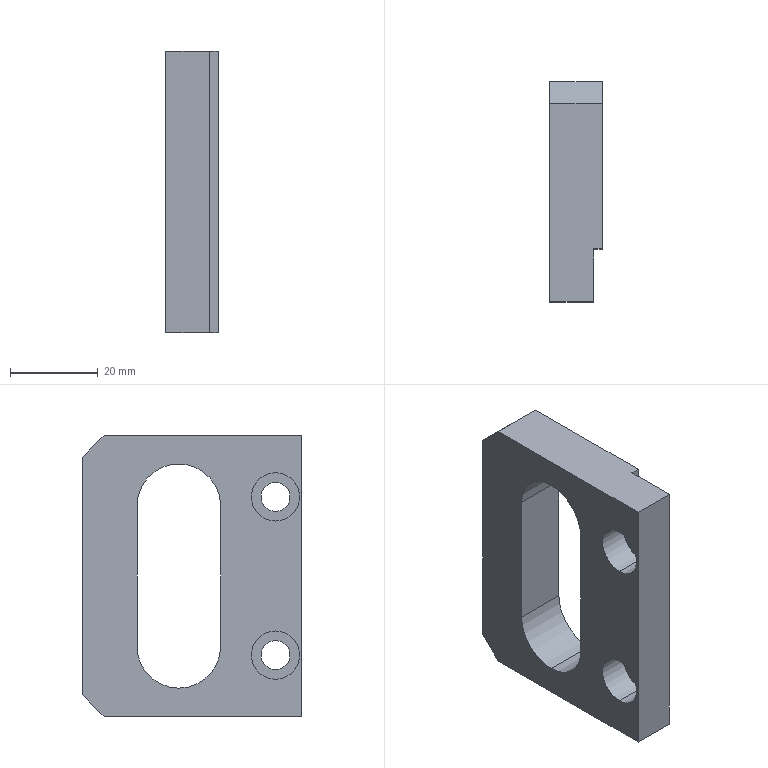Component | SolidWorks | ClampingAssembly-1_A76-1 | 1 solid | 25 faces | box 12 x 50 x 64 mm | volume 24339 mm3 | plane 14 | cylinder 11 | commonest cylinder face diameters 11 x4 6.6 x4 19.02 x3 | material S136
build123d program:
from build123d import *

# Parameters (mm, degrees)
SKETCH1_W                                          = 64
SKETCH1_H                                          = 50
BOSS_EXTRUDE1_DEPTH                                = 6
CUT_EXTRUDE1_DEPTH                                 = 43.344
CHAMFER1_SIZE                                      = 5
SKETCH3_W                                          = 64
SKETCH3_H                                          = 12
CUT_EXTRUDE2_DEPTH                                 = 2
HOLE_SIZE_ACCORDING_TO_TYPE_1_OF_HEXAG_D           = 6.6
HOLE_SIZE_ACCORDING_TO_TYPE_1_OF_HEXAG_CBORE_D     = 11
HOLE_SIZE_ACCORDING_TO_TYPE_1_OF_HEXAG_CBORE_DEPTH = 6.8


with BuildPart() as part:
    # Sketch1 → Boss-Extrude1 (new, symmetric)
    with BuildSketch(Plane(origin=(0, 0, 0), x_dir=(0, 0, -1), z_dir=(1, 0, 0))):
        Rectangle(SKETCH1_W, SKETCH1_H)
    extrude(amount=BOSS_EXTRUDE1_DEPTH, both=True)

    # Sketch2 → Cut-Extrude1 (cut, through all)
    with BuildSketch(Plane(origin=(6, 0, 0), x_dir=(0, 0, -1), z_dir=(1, 0, 0))):
        with BuildLine():
            Line((-16, 12.51), (16, 12.51))
            ThreePointArc((16, 12.51), (25.51, 3), (16, -6.51))
            Line((16, -6.51), (-16, -6.51))
            ThreePointArc((-16, -6.51), (-25.51, 3), (-16, 12.51))
        make_face()
    extrude(amount=-CUT_EXTRUDE1_DEPTH, mode=Mode.SUBTRACT)

    # Chamfer1
    chamfer1_edges = [part.edges().sort_by_distance(p)[0] for p in [
        (0, 25, 32),
        (0, 25, -32),
    ]]
    chamfer(chamfer1_edges, length=CHAMFER1_SIZE)

    # Sketch3 → Cut-Extrude2 (cut)
    with BuildSketch(Plane(origin=(6, 0, 0), x_dir=(0, 0, -1), z_dir=(1, 0, 0))):
        with Locations((0, -19)):
            Rectangle(SKETCH3_W, SKETCH3_H)
    extrude(amount=-CUT_EXTRUDE2_DEPTH, mode=Mode.SUBTRACT)

    # Hole Size _According to_ Type 1 of Hexag (through all)
    with Locations(Plane.ZY.offset(6)):
        with Locations((-18, -19), (18, -19)):
            CounterBoreHole(HOLE_SIZE_ACCORDING_TO_TYPE_1_OF_HEXAG_D / 2, HOLE_SIZE_ACCORDING_TO_TYPE_1_OF_HEXAG_CBORE_D / 2, HOLE_SIZE_ACCORDING_TO_TYPE_1_OF_HEXAG_CBORE_DEPTH)


solid = part.part

# Placed as in the assembly
solid = solid.moved(Location((-8.551, 63.036, -37.5), (0, 0, 0)))
STEP:
#1=COLOUR_RGB('',0.7922,0.8196,0.9333);
#2=FILL_AREA_STYLE_COLOUR('',#1);
#3=FILL_AREA_STYLE('',(#2));
#4=SURFACE_STYLE_FILL_AREA(#3);
#5=SURFACE_SIDE_STYLE('',(#4));
#6=SURFACE_STYLE_USAGE(.BOTH.,#5);
#7=PRESENTATION_STYLE_ASSIGNMENT((#6));
#8=CARTESIAN_POINT('',(-0.3051,1.734,-2.402));
#9=VERTEX_POINT('',#8);
#10=CARTESIAN_POINT('',(-0.3051,1.734,-1.969));
#11=VERTEX_POINT('',#10);
#12=CARTESIAN_POINT('',(-0.3051,1.734,-2.185));
#13=DIRECTION('',(-1.,0.,0.));
#14=DIRECTION('',(0.,0.,1.));
#15=AXIS2_PLACEMENT_3D('',#12,#13,#14);
#16=CIRCLE('',#15,0.2165);
#17=EDGE_CURVE('',#9,#11,#16,.T.);
#18=ORIENTED_EDGE('',*,*,#17,.F.);
#19=CARTESIAN_POINT('',(-0.5729,1.734,-2.402));
#20=VERTEX_POINT('',#19);
#21=CARTESIAN_POINT('',(-0.5729,1.734,-2.402));
#22=DIRECTION('',(-1.,0.,0.));
#23=VECTOR('',#22,39.37);
#24=LINE('',#21,#23);
#25=EDGE_CURVE('',#9,#20,#24,.T.);
#26=ORIENTED_EDGE('',*,*,#25,.T.);
#27=CARTESIAN_POINT('',(-0.5729,1.734,-1.969));
#28=VERTEX_POINT('',#27);
#29=CARTESIAN_POINT('',(-0.5729,1.734,-2.185));
#30=DIRECTION('',(-1.,0.,0.));
#31=DIRECTION('',(0.,0.,1.));
#32=AXIS2_PLACEMENT_3D('',#29,#30,#31);
#33=CIRCLE('',#32,0.2165);
#34=EDGE_CURVE('',#20,#28,#33,.T.);
#35=ORIENTED_EDGE('',*,*,#34,.T.);
#36=CARTESIAN_POINT('',(-0.5729,1.734,-1.969));
#37=DIRECTION('',(-1.,0.,0.));
#38=VECTOR('',#37,39.37);
#39=LINE('',#36,#38);
#40=EDGE_CURVE('',#11,#28,#39,.T.);
#41=ORIENTED_EDGE('',*,*,#40,.F.);
#42=EDGE_LOOP('',(#18,#26,#35,#41));
#43=FACE_OUTER_BOUND('',#42,.T.);
#44=CARTESIAN_POINT('',(-0.5729,1.734,-2.185));
#45=DIRECTION('',(-1.,0.,0.));
#46=DIRECTION('',(0.,0.,1.));
#47=AXIS2_PLACEMENT_3D('',#44,#45,#46);
#48=CYLINDRICAL_SURFACE('',#47,0.2165);
#49=ADVANCED_FACE('',(#43),#48,.F.);
#50=CARTESIAN_POINT('',(-0.1792,1.734,-2.315));
#51=VERTEX_POINT('',#50);
#52=CARTESIAN_POINT('',(-0.1792,1.734,-2.055));
#53=VERTEX_POINT('',#52);
#54=CARTESIAN_POINT('',(-0.1792,1.734,-2.185));
#55=DIRECTION('',(-1.,0.,0.));
#56=DIRECTION('',(0.,0.,1.));
#57=AXIS2_PLACEMENT_3D('',#54,#55,#56);
#58=CIRCLE('',#57,0.1299);
#59=EDGE_CURVE('',#51,#53,#58,.T.);
#60=ORIENTED_EDGE('',*,*,#59,.F.);
#61=CARTESIAN_POINT('',(-0.3051,1.734,-2.315));
#62=VERTEX_POINT('',#61);
#63=CARTESIAN_POINT('',(-0.5729,1.734,-2.315));
#64=DIRECTION('',(-1.,0.,0.));
#65=VECTOR('',#64,39.37);
#66=LINE('',#63,#65);
#67=EDGE_CURVE('',#51,#62,#66,.T.);
#68=ORIENTED_EDGE('',*,*,#67,.T.);
#69=CARTESIAN_POINT('',(-0.3051,1.734,-2.055));
#70=VERTEX_POINT('',#69);
#71=CARTESIAN_POINT('',(-0.3051,1.734,-2.185));
#72=DIRECTION('',(-1.,0.,0.));
#73=DIRECTION('',(0.,0.,1.));
#74=AXIS2_PLACEMENT_3D('',#71,#72,#73);
#75=CIRCLE('',#74,0.1299);
#76=EDGE_CURVE('',#62,#70,#75,.T.);
#77=ORIENTED_EDGE('',*,*,#76,.T.);
#78=CARTESIAN_POINT('',(-0.5729,1.734,-2.055));
#79=DIRECTION('',(-1.,0.,0.));
#80=VECTOR('',#79,39.37);
#81=LINE('',#78,#80);
#82=EDGE_CURVE('',#53,#70,#81,.T.);
#83=ORIENTED_EDGE('',*,*,#82,.F.);
#84=EDGE_LOOP('',(#60,#68,#77,#83));
#85=FACE_OUTER_BOUND('',#84,.T.);
#86=CARTESIAN_POINT('',(-0.5729,1.734,-2.185));
#87=DIRECTION('',(-1.,0.,0.));
#88=DIRECTION('',(0.,0.,1.));
#89=AXIS2_PLACEMENT_3D('',#86,#87,#88);
#90=CYLINDRICAL_SURFACE('',#89,0.1299);
#91=ADVANCED_FACE('',(#85),#90,.F.);
#92=CARTESIAN_POINT('',(-0.3051,1.734,-0.9843));
#93=VERTEX_POINT('',#92);
#94=CARTESIAN_POINT('',(-0.3051,1.734,-0.5512));
#95=VERTEX_POINT('',#94);
#96=CARTESIAN_POINT('',(-0.3051,1.734,-0.7677));
#97=DIRECTION('',(-1.,0.,0.));
#98=DIRECTION('',(0.,0.,1.));
#99=AXIS2_PLACEMENT_3D('',#96,#97,#98);
#100=CIRCLE('',#99,0.2165);
#101=EDGE_CURVE('',#93,#95,#100,.T.);
#102=ORIENTED_EDGE('',*,*,#101,.F.);
#103=CARTESIAN_POINT('',(-0.5729,1.734,-0.9843));
#104=VERTEX_POINT('',#103);
#105=CARTESIAN_POINT('',(-0.5729,1.734,-0.9843));
#106=DIRECTION('',(-1.,0.,0.));
#107=VECTOR('',#106,39.37);
#108=LINE('',#105,#107);
#109=EDGE_CURVE('',#93,#104,#108,.T.);
#110=ORIENTED_EDGE('',*,*,#109,.T.);
#111=CARTESIAN_POINT('',(-0.5729,1.734,-0.5512));
#112=VERTEX_POINT('',#111);
#113=CARTESIAN_POINT('',(-0.5729,1.734,-0.7677));
#114=DIRECTION('',(-1.,0.,0.));
#115=DIRECTION('',(0.,0.,1.));
#116=AXIS2_PLACEMENT_3D('',#113,#114,#115);
#117=CIRCLE('',#116,0.2165);
#118=EDGE_CURVE('',#104,#112,#117,.T.);
#119=ORIENTED_EDGE('',*,*,#118,.T.);
#120=CARTESIAN_POINT('',(-0.5729,1.734,-0.5512));
#121=DIRECTION('',(-1.,0.,0.));
#122=VECTOR('',#121,39.37);
#123=LINE('',#120,#122);
#124=EDGE_CURVE('',#95,#112,#123,.T.);
#125=ORIENTED_EDGE('',*,*,#124,.F.);
#126=EDGE_LOOP('',(#102,#110,#119,#125));
#127=FACE_OUTER_BOUND('',#126,.T.);
#128=CARTESIAN_POINT('',(-0.5729,1.734,-0.7677));
#129=DIRECTION('',(-1.,0.,0.));
#130=DIRECTION('',(0.,0.,1.));
#131=AXIS2_PLACEMENT_3D('',#128,#129,#130);
#132=CYLINDRICAL_SURFACE('',#131,0.2165);
#133=ADVANCED_FACE('',(#127),#132,.F.);
#134=CARTESIAN_POINT('',(-0.1792,1.734,-0.8976));
#135=VERTEX_POINT('',#134);
#136=CARTESIAN_POINT('',(-0.1792,1.734,-0.6378));
#137=VERTEX_POINT('',#136);
#138=CARTESIAN_POINT('',(-0.1792,1.734,-0.7677));
#139=DIRECTION('',(-1.,0.,0.));
#140=DIRECTION('',(0.,0.,1.));
#141=AXIS2_PLACEMENT_3D('',#138,#139,#140);
#142=CIRCLE('',#141,0.1299);
#143=EDGE_CURVE('',#135,#137,#142,.T.);
#144=ORIENTED_EDGE('',*,*,#143,.F.);
#145=CARTESIAN_POINT('',(-0.3051,1.734,-0.8976));
#146=VERTEX_POINT('',#145);
#147=CARTESIAN_POINT('',(-0.5729,1.734,-0.8976));
#148=DIRECTION('',(-1.,0.,0.));
#149=VECTOR('',#148,39.37);
#150=LINE('',#147,#149);
#151=EDGE_CURVE('',#135,#146,#150,.T.);
#152=ORIENTED_EDGE('',*,*,#151,.T.);
#153=CARTESIAN_POINT('',(-0.3051,1.734,-0.6378));
#154=VERTEX_POINT('',#153);
#155=CARTESIAN_POINT('',(-0.3051,1.734,-0.7677));
#156=DIRECTION('',(-1.,0.,0.));
#157=DIRECTION('',(0.,0.,1.));
#158=AXIS2_PLACEMENT_3D('',#155,#156,#157);
#159=CIRCLE('',#158,0.1299);
#160=EDGE_CURVE('',#146,#154,#159,.T.);
#161=ORIENTED_EDGE('',*,*,#160,.T.);
#162=CARTESIAN_POINT('',(-0.5729,1.734,-0.6378));
#163=DIRECTION('',(-1.,0.,0.));
#164=VECTOR('',#163,39.37);
#165=LINE('',#162,#164);
#166=EDGE_CURVE('',#137,#154,#165,.T.);
#167=ORIENTED_EDGE('',*,*,#166,.F.);
#168=EDGE_LOOP('',(#144,#152,#161,#167));
#169=FACE_OUTER_BOUND('',#168,.T.);
#170=CARTESIAN_POINT('',(-0.5729,1.734,-0.7677));
#171=DIRECTION('',(-1.,0.,0.));
#172=DIRECTION('',(0.,0.,1.));
#173=AXIS2_PLACEMENT_3D('',#170,#171,#172);
#174=CYLINDRICAL_SURFACE('',#173,0.1299);
#175=ADVANCED_FACE('',(#169),#174,.F.);
#176=CARTESIAN_POINT('',(-0.5729,2.6,-2.481));
#177=VERTEX_POINT('',#176);
#178=CARTESIAN_POINT('',(-0.5729,2.974,-2.106));
#179=VERTEX_POINT('',#178);
#180=CARTESIAN_POINT('',(-0.5729,2.6,-2.106));
#181=DIRECTION('',(1.,0.,0.));
#182=DIRECTION('',(0.,0.,-1.));
#183=AXIS2_PLACEMENT_3D('',#180,#181,#182);
#184=CIRCLE('',#183,0.3744);
#185=EDGE_CURVE('',#177,#179,#184,.T.);
#186=ORIENTED_EDGE('',*,*,#185,.F.);
#187=CARTESIAN_POINT('',(-0.1004,2.6,-2.481));
#188=VERTEX_POINT('',#187);
#189=CARTESIAN_POINT('',(-0.5729,2.6,-2.481));
#190=DIRECTION('',(1.,0.,0.));
#191=VECTOR('',#190,39.37);
#192=LINE('',#189,#191);
#193=EDGE_CURVE('',#177,#188,#192,.T.);
#194=ORIENTED_EDGE('',*,*,#193,.T.);
#195=CARTESIAN_POINT('',(-0.1004,2.974,-2.106));
#196=VERTEX_POINT('',#195);
#197=CARTESIAN_POINT('',(-0.1004,2.6,-2.106));
#198=DIRECTION('',(1.,0.,0.));
#199=DIRECTION('',(0.,0.,-1.));
#200=AXIS2_PLACEMENT_3D('',#197,#198,#199);
#201=CIRCLE('',#200,0.3744);
#202=EDGE_CURVE('',#188,#196,#201,.T.);
#203=ORIENTED_EDGE('',*,*,#202,.T.);
#204=CARTESIAN_POINT('',(-0.5729,2.974,-2.106));
#205=DIRECTION('',(1.,0.,0.));
#206=VECTOR('',#205,39.37);
#207=LINE('',#204,#206);
#208=EDGE_CURVE('',#179,#196,#207,.T.);
#209=ORIENTED_EDGE('',*,*,#208,.F.);
#210=EDGE_LOOP('',(#186,#194,#203,#209));
#211=FACE_OUTER_BOUND('',#210,.T.);
#212=CARTESIAN_POINT('',(-0.5729,2.6,-2.106));
#213=DIRECTION('',(1.,0.,0.));
#214=DIRECTION('',(0.,0.,-1.));
#215=AXIS2_PLACEMENT_3D('',#212,#213,#214);
#216=CYLINDRICAL_SURFACE('',#215,0.3744);
#217=ADVANCED_FACE('',(#211),#216,.F.);
#218=CARTESIAN_POINT('',(-0.1004,1.97,-2.736));
#219=VERTEX_POINT('',#218);
#220=CARTESIAN_POINT('',(-0.1004,3.269,-2.736));
#221=VERTEX_POINT('',#220);
#222=CARTESIAN_POINT('',(-0.1004,3.466,-2.736));
#223=DIRECTION('',(0.,1.,0.));
#224=VECTOR('',#223,39.37);
#225=LINE('',#222,#224);
#226=EDGE_CURVE('',#219,#221,#225,.T.);
#227=ORIENTED_EDGE('',*,*,#226,.F.);
#228=CARTESIAN_POINT('',(-0.1792,1.97,-2.736));
#229=VERTEX_POINT('',#228);
#230=CARTESIAN_POINT('',(-0.1792,1.97,-2.736));
#231=DIRECTION('',(1.,0.,0.));
#232=VECTOR('',#231,39.37);
#233=LINE('',#230,#232);
#234=EDGE_CURVE('',#229,#219,#233,.T.);
#235=ORIENTED_EDGE('',*,*,#234,.F.);
#236=CARTESIAN_POINT('',(-0.1792,1.497,-2.736));
#237=VERTEX_POINT('',#236);
#238=CARTESIAN_POINT('',(-0.1792,1.497,-2.736));
#239=DIRECTION('',(0.,1.,0.));
#240=VECTOR('',#239,39.37);
#241=LINE('',#238,#240);
#242=EDGE_CURVE('',#237,#229,#241,.T.);
#243=ORIENTED_EDGE('',*,*,#242,.F.);
#244=CARTESIAN_POINT('',(-0.5729,1.497,-2.736));
#245=VERTEX_POINT('',#244);
#246=CARTESIAN_POINT('',(-0.1004,1.497,-2.736));
#247=DIRECTION('',(-1.,0.,0.));
#248=VECTOR('',#247,39.37);
#249=LINE('',#246,#248);
#250=EDGE_CURVE('',#237,#245,#249,.T.);
#251=ORIENTED_EDGE('',*,*,#250,.T.);
#252=CARTESIAN_POINT('',(-0.5729,3.269,-2.736));
#253=VERTEX_POINT('',#252);
#254=CARTESIAN_POINT('',(-0.5729,3.466,-2.736));
#255=DIRECTION('',(0.,1.,0.));
#256=VECTOR('',#255,39.37);
#257=LINE('',#254,#256);
#258=EDGE_CURVE('',#245,#253,#257,.T.);
#259=ORIENTED_EDGE('',*,*,#258,.T.);
#260=CARTESIAN_POINT('',(-0.1004,3.269,-2.736));
#261=DIRECTION('',(1.,0.,0.));
#262=VECTOR('',#261,39.37);
#263=LINE('',#260,#262);
#264=EDGE_CURVE('',#253,#221,#263,.T.);
#265=ORIENTED_EDGE('',*,*,#264,.T.);
#266=EDGE_LOOP('',(#227,#235,#243,#251,#259,#265));
#267=FACE_OUTER_BOUND('',#266,.T.);
#268=CARTESIAN_POINT('',(-0.1004,3.466,-2.736));
#269=DIRECTION('',(0.,0.,1.));
#270=DIRECTION('',(1.,0.,0.));
#271=AXIS2_PLACEMENT_3D('',#268,#269,#270);
#272=PLANE('',#271);
#273=ADVANCED_FACE('',(#267),#272,.F.);
#274=CARTESIAN_POINT('',(-0.5729,3.466,-2.539));
#275=VERTEX_POINT('',#274);
#276=CARTESIAN_POINT('',(-0.5729,3.466,-0.4134));
#277=VERTEX_POINT('',#276);
#278=CARTESIAN_POINT('',(-0.5729,3.466,-0.2165));
#279=DIRECTION('',(0.,0.,1.));
#280=VECTOR('',#279,39.37);
#281=LINE('',#278,#280);
#282=EDGE_CURVE('',#275,#277,#281,.T.);
#283=ORIENTED_EDGE('',*,*,#282,.T.);
#284=CARTESIAN_POINT('',(-0.1004,3.466,-0.4134));
#285=VERTEX_POINT('',#284);
#286=CARTESIAN_POINT('',(-0.1004,3.466,-0.4134));
#287=DIRECTION('',(1.,0.,0.));
#288=VECTOR('',#287,39.37);
#289=LINE('',#286,#288);
#290=EDGE_CURVE('',#277,#285,#289,.T.);
#291=ORIENTED_EDGE('',*,*,#290,.T.);
#292=CARTESIAN_POINT('',(-0.1004,3.466,-2.539));
#293=VERTEX_POINT('',#292);
#294=CARTESIAN_POINT('',(-0.1004,3.466,-0.2165));
#295=DIRECTION('',(0.,0.,1.));
#296=VECTOR('',#295,39.37);
#297=LINE('',#294,#296);
#298=EDGE_CURVE('',#293,#285,#297,.T.);
#299=ORIENTED_EDGE('',*,*,#298,.F.);
#300=CARTESIAN_POINT('',(-0.1004,3.466,-2.539));
#301=DIRECTION('',(-1.,0.,0.));
#302=VECTOR('',#301,39.37);
#303=LINE('',#300,#302);
#304=EDGE_CURVE('',#293,#275,#303,.T.);
#305=ORIENTED_EDGE('',*,*,#304,.T.);
#306=EDGE_LOOP('',(#283,#291,#299,#305));
#307=FACE_OUTER_BOUND('',#306,.T.);
#308=CARTESIAN_POINT('',(-0.1004,3.466,-0.2165));
#309=DIRECTION('',(0.,-1.,0.));
#310=DIRECTION('',(0.,0.,-1.));
#311=AXIS2_PLACEMENT_3D('',#308,#309,#310);
#312=PLANE('',#311);
#313=ADVANCED_FACE('',(#307),#312,.F.);
#314=CARTESIAN_POINT('',(-0.1792,1.97,-0.2165));
#315=VERTEX_POINT('',#314);
#316=CARTESIAN_POINT('',(-0.1792,1.497,-0.2165));
#317=VERTEX_POINT('',#316);
#318=CARTESIAN_POINT('',(-0.1792,1.497,-0.2165));
#319=DIRECTION('',(0.,-1.,0.));
#320=VECTOR('',#319,39.37);
#321=LINE('',#318,#320);
#322=EDGE_CURVE('',#315,#317,#321,.T.);
#323=ORIENTED_EDGE('',*,*,#322,.F.);
#324=CARTESIAN_POINT('',(-0.1004,1.97,-0.2165));
#325=VERTEX_POINT('',#324);
#326=CARTESIAN_POINT('',(-0.1792,1.97,-0.2165));
#327=DIRECTION('',(1.,0.,0.));
#328=VECTOR('',#327,39.37);
#329=LINE('',#326,#328);
#330=EDGE_CURVE('',#315,#325,#329,.T.);
#331=ORIENTED_EDGE('',*,*,#330,.T.);
#332=CARTESIAN_POINT('',(-0.1004,3.269,-0.2165));
#333=VERTEX_POINT('',#332);
#334=CARTESIAN_POINT('',(-0.1004,3.466,-0.2165));
#335=DIRECTION('',(0.,-1.,-0.));
#336=VECTOR('',#335,39.37);
#337=LINE('',#334,#336);
#338=EDGE_CURVE('',#333,#325,#337,.T.);
#339=ORIENTED_EDGE('',*,*,#338,.F.);
#340=CARTESIAN_POINT('',(-0.5729,3.269,-0.2165));
#341=VERTEX_POINT('',#340);
#342=CARTESIAN_POINT('',(-0.1004,3.269,-0.2165));
#343=DIRECTION('',(-1.,0.,0.));
#344=VECTOR('',#343,39.37);
#345=LINE('',#342,#344);
#346=EDGE_CURVE('',#333,#341,#345,.T.);
#347=ORIENTED_EDGE('',*,*,#346,.T.);
#348=CARTESIAN_POINT('',(-0.5729,1.497,-0.2165));
#349=VERTEX_POINT('',#348);
#350=CARTESIAN_POINT('',(-0.5729,3.466,-0.2165));
#351=DIRECTION('',(0.,-1.,-0.));
#352=VECTOR('',#351,39.37);
#353=LINE('',#350,#352);
#354=EDGE_CURVE('',#341,#349,#353,.T.);
#355=ORIENTED_EDGE('',*,*,#354,.T.);
#356=CARTESIAN_POINT('',(-0.1004,1.497,-0.2165));
#357=DIRECTION('',(-1.,0.,0.));
#358=VECTOR('',#357,39.37);
#359=LINE('',#356,#358);
#360=EDGE_CURVE('',#317,#349,#359,.T.);
#361=ORIENTED_EDGE('',*,*,#360,.F.);
#362=EDGE_LOOP('',(#323,#331,#339,#347,#355,#361));
#363=FACE_OUTER_BOUND('',#362,.T.);
#364=CARTESIAN_POINT('',(-0.1004,3.466,-0.2165));
#365=DIRECTION('',(0.,0.,-1.));
#366=DIRECTION('',(0.,1.,0.));
#367=AXIS2_PLACEMENT_3D('',#364,#365,#366);
#368=PLANE('',#367);
#369=ADVANCED_FACE('',(#363),#368,.F.);
#370=ORIENTED_EDGE('',*,*,#250,.F.);
#371=CARTESIAN_POINT('',(-0.1792,1.497,-0.2165));
#372=DIRECTION('',(0.,0.,-1.));
#373=VECTOR('',#372,39.37);
#374=LINE('',#371,#373);
#375=EDGE_CURVE('',#317,#237,#374,.T.);
#376=ORIENTED_EDGE('',*,*,#375,.F.);
#377=ORIENTED_EDGE('',*,*,#360,.T.);
#378=CARTESIAN_POINT('',(-0.5729,1.497,-0.2165));
#379=DIRECTION('',(0.,0.,-1.));
#380=VECTOR('',#379,39.37);
#381=LINE('',#378,#380);
#382=EDGE_CURVE('',#349,#245,#381,.T.);
#383=ORIENTED_EDGE('',*,*,#382,.T.);
#384=EDGE_LOOP('',(#370,#376,#377,#383));
#385=FACE_OUTER_BOUND('',#384,.T.);
#386=CARTESIAN_POINT('',(-0.1004,1.497,-0.2165));
#387=DIRECTION('',(0.,1.,0.));
#388=DIRECTION('',(0.,0.,1.));
#389=AXIS2_PLACEMENT_3D('',#386,#387,#388);
#390=PLANE('',#389);
#391=ADVANCED_FACE('',(#385),#390,.F.);
#392=CARTESIAN_POINT('',(-0.1004,1.97,-0.2165));
#393=DIRECTION('',(0.,0.,1.));
#394=VECTOR('',#393,39.37);
#395=LINE('',#392,#394);
#396=EDGE_CURVE('',#219,#325,#395,.T.);
#397=ORIENTED_EDGE('',*,*,#396,.F.);
#398=ORIENTED_EDGE('',*,*,#226,.T.);
#399=CARTESIAN_POINT('',(-0.1004,3.505,-2.5));
#400=DIRECTION('',(0.,0.7071,0.7071));
#401=VECTOR('',#400,39.37);
#402=LINE('',#399,#401);
#403=EDGE_CURVE('',#221,#293,#402,.T.);
#404=ORIENTED_EDGE('',*,*,#403,.T.);
#405=ORIENTED_EDGE('',*,*,#298,.T.);
#406=CARTESIAN_POINT('',(-0.1004,3.505,-0.4528));
#407=DIRECTION('',(0.,-0.7071,0.7071));
#408=VECTOR('',#407,39.37);
#409=LINE('',#406,#408);
#410=EDGE_CURVE('',#285,#333,#409,.T.);
#411=ORIENTED_EDGE('',*,*,#410,.T.);
#412=ORIENTED_EDGE('',*,*,#338,.T.);
#413=EDGE_LOOP('',(#397,#398,#404,#405,#411,#412));
#414=FACE_OUTER_BOUND('',#413,.T.);
#415=CARTESIAN_POINT('',(-0.1004,2.974,-0.8465));
#416=VERTEX_POINT('',#415);
#417=CARTESIAN_POINT('',(-0.1004,2.225,-0.8465));
#418=VERTEX_POINT('',#417);
#419=CARTESIAN_POINT('',(-0.1004,2.6,-0.8465));
#420=DIRECTION('',(1.,0.,0.));
#421=DIRECTION('',(0.,0.,-1.));
#422=AXIS2_PLACEMENT_3D('',#419,#420,#421);
#423=CIRCLE('',#422,0.3744);
#424=EDGE_CURVE('',#416,#418,#423,.T.);
#425=ORIENTED_EDGE('',*,*,#424,.F.);
#426=CARTESIAN_POINT('',(-0.1004,2.974,-0.8465));
#427=DIRECTION('',(0.,0.,1.));
#428=VECTOR('',#427,39.37);
#429=LINE('',#426,#428);
#430=EDGE_CURVE('',#196,#416,#429,.T.);
#431=ORIENTED_EDGE('',*,*,#430,.F.);
#432=ORIENTED_EDGE('',*,*,#202,.F.);
#433=CARTESIAN_POINT('',(-0.1004,2.225,-2.106));
#434=VERTEX_POINT('',#433);
#435=CARTESIAN_POINT('',(-0.1004,2.6,-2.106));
#436=DIRECTION('',(1.,0.,0.));
#437=DIRECTION('',(0.,0.,-1.));
#438=AXIS2_PLACEMENT_3D('',#435,#436,#437);
#439=CIRCLE('',#438,0.3744);
#440=EDGE_CURVE('',#434,#188,#439,.T.);
#441=ORIENTED_EDGE('',*,*,#440,.F.);
#442=CARTESIAN_POINT('',(-0.1004,2.225,-0.8465));
#443=DIRECTION('',(0.,0.,-1.));
#444=VECTOR('',#443,39.37);
#445=LINE('',#442,#444);
#446=EDGE_CURVE('',#418,#434,#445,.T.);
#447=ORIENTED_EDGE('',*,*,#446,.F.);
#448=EDGE_LOOP('',(#425,#431,#432,#441,#447));
#449=FACE_BOUND('',#448,.T.);
#450=CARTESIAN_POINT('',(-0.1004,2.482,-1.476));
#451=DIRECTION('',(1.,0.,0.));
#452=DIRECTION('',(0.,0.,-1.));
#453=AXIS2_PLACEMENT_3D('',#450,#451,#452);
#454=PLANE('',#453);
#455=ADVANCED_FACE('',(#414,#449),#454,.T.);
#456=CARTESIAN_POINT('',(-0.5729,1.734,-2.185));
#457=DIRECTION('',(-1.,0.,0.));
#458=DIRECTION('',(0.,0.,1.));
#459=AXIS2_PLACEMENT_3D('',#456,#457,#458);
#460=CIRCLE('',#459,0.2165);
#461=EDGE_CURVE('',#28,#20,#460,.T.);
#462=ORIENTED_EDGE('',*,*,#461,.F.);
#463=ORIENTED_EDGE('',*,*,#34,.F.);
#464=EDGE_LOOP('',(#462,#463));
#465=FACE_BOUND('',#464,.T.);
#466=CARTESIAN_POINT('',(-0.5729,1.734,-0.7677));
#467=DIRECTION('',(-1.,0.,0.));
#468=DIRECTION('',(0.,0.,1.));
#469=AXIS2_PLACEMENT_3D('',#466,#467,#468);
#470=CIRCLE('',#469,0.2165);
#471=EDGE_CURVE('',#112,#104,#470,.T.);
#472=ORIENTED_EDGE('',*,*,#471,.F.);
#473=ORIENTED_EDGE('',*,*,#118,.F.);
#474=EDGE_LOOP('',(#472,#473));
#475=FACE_BOUND('',#474,.T.);
#476=CARTESIAN_POINT('',(-0.5729,2.974,-0.8465));
#477=VERTEX_POINT('',#476);
#478=CARTESIAN_POINT('',(-0.5729,2.974,-0.8465));
#479=DIRECTION('',(0.,0.,1.));
#480=VECTOR('',#479,39.37);
#481=LINE('',#478,#480);
#482=EDGE_CURVE('',#179,#477,#481,.T.);
#483=ORIENTED_EDGE('',*,*,#482,.T.);
#484=CARTESIAN_POINT('',(-0.5729,2.225,-0.8465));
#485=VERTEX_POINT('',#484);
#486=CARTESIAN_POINT('',(-0.5729,2.6,-0.8465));
#487=DIRECTION('',(1.,0.,0.));
#488=DIRECTION('',(0.,0.,-1.));
#489=AXIS2_PLACEMENT_3D('',#486,#487,#488);
#490=CIRCLE('',#489,0.3744);
#491=EDGE_CURVE('',#477,#485,#490,.T.);
#492=ORIENTED_EDGE('',*,*,#491,.T.);
#493=CARTESIAN_POINT('',(-0.5729,2.225,-2.106));
#494=VERTEX_POINT('',#493);
#495=CARTESIAN_POINT('',(-0.5729,2.225,-0.8465));
#496=DIRECTION('',(0.,0.,-1.));
#497=VECTOR('',#496,39.37);
#498=LINE('',#495,#497);
#499=EDGE_CURVE('',#485,#494,#498,.T.);
#500=ORIENTED_EDGE('',*,*,#499,.T.);
#501=CARTESIAN_POINT('',(-0.5729,2.6,-2.106));
#502=DIRECTION('',(1.,0.,0.));
#503=DIRECTION('',(0.,0.,-1.));
#504=AXIS2_PLACEMENT_3D('',#501,#502,#503);
#505=CIRCLE('',#504,0.3744);
#506=EDGE_CURVE('',#494,#177,#505,.T.);
#507=ORIENTED_EDGE('',*,*,#506,.T.);
#508=ORIENTED_EDGE('',*,*,#185,.T.);
#509=EDGE_LOOP('',(#483,#492,#500,#507,#508));
#510=FACE_BOUND('',#509,.T.);
#511=ORIENTED_EDGE('',*,*,#354,.F.);
#512=CARTESIAN_POINT('',(-0.5729,3.269,-0.2165));
#513=DIRECTION('',(0.,0.7071,-0.7071));
#514=VECTOR('',#513,39.37);
#515=LINE('',#512,#514);
#516=EDGE_CURVE('',#341,#277,#515,.T.);
#517=ORIENTED_EDGE('',*,*,#516,.T.);
#518=ORIENTED_EDGE('',*,*,#282,.F.);
#519=CARTESIAN_POINT('',(-0.5729,3.466,-2.539));
#520=DIRECTION('',(0.,-0.7071,-0.7071));
#521=VECTOR('',#520,39.37);
#522=LINE('',#519,#521);
#523=EDGE_CURVE('',#275,#253,#522,.T.);
#524=ORIENTED_EDGE('',*,*,#523,.T.);
#525=ORIENTED_EDGE('',*,*,#258,.F.);
#526=ORIENTED_EDGE('',*,*,#382,.F.);
#527=EDGE_LOOP('',(#511,#517,#518,#524,#525,#526));
#528=FACE_OUTER_BOUND('',#527,.T.);
#529=CARTESIAN_POINT('',(-0.5729,2.482,-1.476));
#530=DIRECTION('',(1.,0.,0.));
#531=DIRECTION('',(0.,0.,-1.));
#532=AXIS2_PLACEMENT_3D('',#529,#530,#531);
#533=PLANE('',#532);
#534=ADVANCED_FACE('',(#465,#475,#510,#528),#533,.F.);
#535=ORIENTED_EDGE('',*,*,#424,.T.);
#536=CARTESIAN_POINT('',(-0.5729,2.225,-0.8465));
#537=DIRECTION('',(1.,0.,0.));
#538=VECTOR('',#537,39.37);
#539=LINE('',#536,#538);
#540=EDGE_CURVE('',#485,#418,#539,.T.);
#541=ORIENTED_EDGE('',*,*,#540,.F.);
#542=ORIENTED_EDGE('',*,*,#491,.F.);
#543=CARTESIAN_POINT('',(-0.5729,2.974,-0.8465));
#544=DIRECTION('',(1.,0.,0.));
#545=VECTOR('',#544,39.37);
#546=LINE('',#543,#545);
#547=EDGE_CURVE('',#477,#416,#546,.T.);
#548=ORIENTED_EDGE('',*,*,#547,.T.);
#549=EDGE_LOOP('',(#535,#541,#542,#548));
#550=FACE_OUTER_BOUND('',#549,.T.);
#551=CARTESIAN_POINT('',(-0.5729,2.6,-0.8465));
#552=DIRECTION('',(1.,0.,0.));
#553=DIRECTION('',(0.,0.,-1.));
#554=AXIS2_PLACEMENT_3D('',#551,#552,#553);
#555=CYLINDRICAL_SURFACE('',#554,0.3744);
#556=ADVANCED_FACE('',(#550),#555,.F.);
#557=ORIENTED_EDGE('',*,*,#430,.T.);
#558=ORIENTED_EDGE('',*,*,#547,.F.);
#559=ORIENTED_EDGE('',*,*,#482,.F.);
#560=ORIENTED_EDGE('',*,*,#208,.T.);
#561=EDGE_LOOP('',(#557,#558,#559,#560));
#562=FACE_OUTER_BOUND('',#561,.T.);
#563=CARTESIAN_POINT('',(-0.5729,2.974,-0.8465));
#564=DIRECTION('',(0.,1.,0.));
#565=DIRECTION('',(0.,0.,1.));
#566=AXIS2_PLACEMENT_3D('',#563,#564,#565);
#567=PLANE('',#566);
#568=ADVANCED_FACE('',(#562),#567,.F.);
#569=ORIENTED_EDGE('',*,*,#193,.F.);
#570=ORIENTED_EDGE('',*,*,#506,.F.);
#571=CARTESIAN_POINT('',(-0.5729,2.225,-2.106));
#572=DIRECTION('',(1.,0.,0.));
#573=VECTOR('',#572,39.37);
#574=LINE('',#571,#573);
#575=EDGE_CURVE('',#494,#434,#574,.T.);
#576=ORIENTED_EDGE('',*,*,#575,.T.);
#577=ORIENTED_EDGE('',*,*,#440,.T.);
#578=EDGE_LOOP('',(#569,#570,#576,#577));
#579=FACE_OUTER_BOUND('',#578,.T.);
#580=CARTESIAN_POINT('',(-0.5729,2.6,-2.106));
#581=DIRECTION('',(1.,0.,0.));
#582=DIRECTION('',(0.,0.,-1.));
#583=AXIS2_PLACEMENT_3D('',#580,#581,#582);
#584=CYLINDRICAL_SURFACE('',#583,0.3744);
#585=ADVANCED_FACE('',(#579),#584,.F.);
#586=ORIENTED_EDGE('',*,*,#446,.T.);
#587=ORIENTED_EDGE('',*,*,#575,.F.);
#588=ORIENTED_EDGE('',*,*,#499,.F.);
#589=ORIENTED_EDGE('',*,*,#540,.T.);
#590=EDGE_LOOP('',(#586,#587,#588,#589));
#591=FACE_OUTER_BOUND('',#590,.T.);
#592=CARTESIAN_POINT('',(-0.5729,2.225,-0.8465));
#593=DIRECTION('',(0.,-1.,0.));
#594=DIRECTION('',(0.,0.,-1.));
#595=AXIS2_PLACEMENT_3D('',#592,#593,#594);
#596=PLANE('',#595);
#597=ADVANCED_FACE('',(#591),#596,.F.);
#598=ORIENTED_EDGE('',*,*,#410,.F.);
#599=ORIENTED_EDGE('',*,*,#290,.F.);
#600=ORIENTED_EDGE('',*,*,#516,.F.);
#601=ORIENTED_EDGE('',*,*,#346,.F.);
#602=EDGE_LOOP('',(#598,#599,#600,#601));
#603=FACE_OUTER_BOUND('',#602,.T.);
#604=CARTESIAN_POINT('',(-0.1004,3.269,-0.2165));
#605=DIRECTION('',(0.,-0.7071,-0.7071));
#606=DIRECTION('',(-1.,0.,0.));
#607=AXIS2_PLACEMENT_3D('',#604,#605,#606);
#608=PLANE('',#607);
#609=ADVANCED_FACE('',(#603),#608,.F.);
#610=ORIENTED_EDGE('',*,*,#403,.F.);
#611=ORIENTED_EDGE('',*,*,#264,.F.);
#612=ORIENTED_EDGE('',*,*,#523,.F.);
#613=ORIENTED_EDGE('',*,*,#304,.F.);
#614=EDGE_LOOP('',(#610,#611,#612,#613));
#615=FACE_OUTER_BOUND('',#614,.T.);
#616=CARTESIAN_POINT('',(-0.1004,3.466,-2.539));
#617=DIRECTION('',(0.,-0.7071,0.7071));
#618=DIRECTION('',(-1.,0.,0.));
#619=AXIS2_PLACEMENT_3D('',#616,#617,#618);
#620=PLANE('',#619);
#621=ADVANCED_FACE('',(#615),#620,.F.);
#622=ORIENTED_EDGE('',*,*,#396,.T.);
#623=ORIENTED_EDGE('',*,*,#330,.F.);
#624=CARTESIAN_POINT('',(-0.1792,1.97,-0.2165));
#625=DIRECTION('',(0.,0.,1.));
#626=VECTOR('',#625,39.37);
#627=LINE('',#624,#626);
#628=EDGE_CURVE('',#229,#315,#627,.T.);
#629=ORIENTED_EDGE('',*,*,#628,.F.);
#630=ORIENTED_EDGE('',*,*,#234,.T.);
#631=EDGE_LOOP('',(#622,#623,#629,#630));
#632=FACE_OUTER_BOUND('',#631,.T.);
#633=CARTESIAN_POINT('',(-0.1792,1.97,-0.2165));
#634=DIRECTION('',(0.,1.,0.));
#635=DIRECTION('',(0.,0.,1.));
#636=AXIS2_PLACEMENT_3D('',#633,#634,#635);
#637=PLANE('',#636);
#638=ADVANCED_FACE('',(#632),#637,.F.);
#639=CARTESIAN_POINT('',(-0.1792,1.734,-2.185));
#640=DIRECTION('',(-1.,0.,0.));
#641=DIRECTION('',(0.,0.,1.));
#642=AXIS2_PLACEMENT_3D('',#639,#640,#641);
#643=CIRCLE('',#642,0.1299);
#644=EDGE_CURVE('',#53,#51,#643,.T.);
#645=ORIENTED_EDGE('',*,*,#644,.T.);
#646=ORIENTED_EDGE('',*,*,#59,.T.);
#647=EDGE_LOOP('',(#645,#646));
#648=FACE_BOUND('',#647,.T.);
#649=CARTESIAN_POINT('',(-0.1792,1.734,-0.7677));
#650=DIRECTION('',(-1.,0.,0.));
#651=DIRECTION('',(0.,0.,1.));
#652=AXIS2_PLACEMENT_3D('',#649,#650,#651);
#653=CIRCLE('',#652,0.1299);
#654=EDGE_CURVE('',#137,#135,#653,.T.);
#655=ORIENTED_EDGE('',*,*,#654,.T.);
#656=ORIENTED_EDGE('',*,*,#143,.T.);
#657=EDGE_LOOP('',(#655,#656));
#658=FACE_BOUND('',#657,.T.);
#659=ORIENTED_EDGE('',*,*,#322,.T.);
#660=ORIENTED_EDGE('',*,*,#375,.T.);
#661=ORIENTED_EDGE('',*,*,#242,.T.);
#662=ORIENTED_EDGE('',*,*,#628,.T.);
#663=EDGE_LOOP('',(#659,#660,#661,#662));
#664=FACE_OUTER_BOUND('',#663,.T.);
#665=CARTESIAN_POINT('',(-0.1792,2.482,-1.476));
#666=DIRECTION('',(-1.,0.,0.));
#667=DIRECTION('',(0.,0.,1.));
#668=AXIS2_PLACEMENT_3D('',#665,#666,#667);
#669=PLANE('',#668);
#670=ADVANCED_FACE('',(#648,#658,#664),#669,.F.);
#671=ORIENTED_EDGE('',*,*,#151,.F.);
#672=ORIENTED_EDGE('',*,*,#654,.F.);
#673=ORIENTED_EDGE('',*,*,#166,.T.);
#674=CARTESIAN_POINT('',(-0.3051,1.734,-0.7677));
#675=DIRECTION('',(-1.,0.,0.));
#676=DIRECTION('',(0.,0.,1.));
#677=AXIS2_PLACEMENT_3D('',#674,#675,#676);
#678=CIRCLE('',#677,0.1299);
#679=EDGE_CURVE('',#154,#146,#678,.T.);
#680=ORIENTED_EDGE('',*,*,#679,.T.);
#681=EDGE_LOOP('',(#671,#672,#673,#680));
#682=FACE_OUTER_BOUND('',#681,.T.);
#683=CARTESIAN_POINT('',(-0.5729,1.734,-0.7677));
#684=DIRECTION('',(-1.,0.,0.));
#685=DIRECTION('',(0.,0.,1.));
#686=AXIS2_PLACEMENT_3D('',#683,#684,#685);
#687=CYLINDRICAL_SURFACE('',#686,0.1299);
#688=ADVANCED_FACE('',(#682),#687,.F.);
#689=ORIENTED_EDGE('',*,*,#679,.F.);
#690=ORIENTED_EDGE('',*,*,#160,.F.);
#691=EDGE_LOOP('',(#689,#690));
#692=FACE_BOUND('',#691,.T.);
#693=CARTESIAN_POINT('',(-0.3051,1.734,-0.7677));
#694=DIRECTION('',(-1.,0.,0.));
#695=DIRECTION('',(0.,0.,1.));
#696=AXIS2_PLACEMENT_3D('',#693,#694,#695);
#697=CIRCLE('',#696,0.2165);
#698=EDGE_CURVE('',#95,#93,#697,.T.);
#699=ORIENTED_EDGE('',*,*,#698,.T.);
#700=ORIENTED_EDGE('',*,*,#101,.T.);
#701=EDGE_LOOP('',(#699,#700));
#702=FACE_OUTER_BOUND('',#701,.T.);
#703=CARTESIAN_POINT('',(-0.3051,1.864,-0.7677));
#704=DIRECTION('',(1.,0.,0.));
#705=DIRECTION('',(0.,0.,-1.));
#706=AXIS2_PLACEMENT_3D('',#703,#704,#705);
#707=PLANE('',#706);
#708=ADVANCED_FACE('',(#692,#702),#707,.F.);
#709=ORIENTED_EDGE('',*,*,#109,.F.);
#710=ORIENTED_EDGE('',*,*,#698,.F.);
#711=ORIENTED_EDGE('',*,*,#124,.T.);
#712=ORIENTED_EDGE('',*,*,#471,.T.);
#713=EDGE_LOOP('',(#709,#710,#711,#712));
#714=FACE_OUTER_BOUND('',#713,.T.);
#715=CARTESIAN_POINT('',(-0.5729,1.734,-0.7677));
#716=DIRECTION('',(-1.,0.,0.));
#717=DIRECTION('',(0.,0.,1.));
#718=AXIS2_PLACEMENT_3D('',#715,#716,#717);
#719=CYLINDRICAL_SURFACE('',#718,0.2165);
#720=ADVANCED_FACE('',(#714),#719,.F.);
#721=ORIENTED_EDGE('',*,*,#67,.F.);
#722=ORIENTED_EDGE('',*,*,#644,.F.);
#723=ORIENTED_EDGE('',*,*,#82,.T.);
#724=CARTESIAN_POINT('',(-0.3051,1.734,-2.185));
#725=DIRECTION('',(-1.,0.,0.));
#726=DIRECTION('',(0.,0.,1.));
#727=AXIS2_PLACEMENT_3D('',#724,#725,#726);
#728=CIRCLE('',#727,0.1299);
#729=EDGE_CURVE('',#70,#62,#728,.T.);
#730=ORIENTED_EDGE('',*,*,#729,.T.);
#731=EDGE_LOOP('',(#721,#722,#723,#730));
#732=FACE_OUTER_BOUND('',#731,.T.);
#733=CARTESIAN_POINT('',(-0.5729,1.734,-2.185));
#734=DIRECTION('',(-1.,0.,0.));
#735=DIRECTION('',(0.,0.,1.));
#736=AXIS2_PLACEMENT_3D('',#733,#734,#735);
#737=CYLINDRICAL_SURFACE('',#736,0.1299);
#738=ADVANCED_FACE('',(#732),#737,.F.);
#739=ORIENTED_EDGE('',*,*,#729,.F.);
#740=ORIENTED_EDGE('',*,*,#76,.F.);
#741=EDGE_LOOP('',(#739,#740));
#742=FACE_BOUND('',#741,.T.);
#743=CARTESIAN_POINT('',(-0.3051,1.734,-2.185));
#744=DIRECTION('',(-1.,0.,0.));
#745=DIRECTION('',(0.,0.,1.));
#746=AXIS2_PLACEMENT_3D('',#743,#744,#745);
#747=CIRCLE('',#746,0.2165);
#748=EDGE_CURVE('',#11,#9,#747,.T.);
#749=ORIENTED_EDGE('',*,*,#748,.T.);
#750=ORIENTED_EDGE('',*,*,#17,.T.);
#751=EDGE_LOOP('',(#749,#750));
#752=FACE_OUTER_BOUND('',#751,.T.);
#753=CARTESIAN_POINT('',(-0.3051,1.864,-2.185));
#754=DIRECTION('',(1.,0.,0.));
#755=DIRECTION('',(0.,0.,-1.));
#756=AXIS2_PLACEMENT_3D('',#753,#754,#755);
#757=PLANE('',#756);
#758=ADVANCED_FACE('',(#742,#752),#757,.F.);
#759=ORIENTED_EDGE('',*,*,#25,.F.);
#760=ORIENTED_EDGE('',*,*,#748,.F.);
#761=ORIENTED_EDGE('',*,*,#40,.T.);
#762=ORIENTED_EDGE('',*,*,#461,.T.);
#763=EDGE_LOOP('',(#759,#760,#761,#762));
#764=FACE_OUTER_BOUND('',#763,.T.);
#765=CARTESIAN_POINT('',(-0.5729,1.734,-2.185));
#766=DIRECTION('',(-1.,0.,0.));
#767=DIRECTION('',(0.,0.,1.));
#768=AXIS2_PLACEMENT_3D('',#765,#766,#767);
#769=CYLINDRICAL_SURFACE('',#768,0.2165);
#770=ADVANCED_FACE('',(#764),#769,.F.);
#771=CLOSED_SHELL('',(#49,#91,#133,#175,#217,#273,#313,#369,#391,#455,#534,#556,#568,#585,#597,#609,#621,#638,#670,#688,#708,#720,#738,#758,#770));
#772=MANIFOLD_SOLID_BREP('',#771);
#773=STYLED_ITEM('',(#7),#772);
#774=(LENGTH_UNIT()NAMED_UNIT(*)SI_UNIT($,.METRE.));
#775=LENGTH_MEASURE_WITH_UNIT(LENGTH_MEASURE(0.0254),#774);
#776=DIMENSIONAL_EXPONENTS(1.,0.,0.,0.,0.,0.,0.);
#777=(CONVERSION_BASED_UNIT('',#775)LENGTH_UNIT()NAMED_UNIT(#776));
#778=UNCERTAINTY_MEASURE_WITH_UNIT(LENGTH_MEASURE(0.00001),#777,'','');
#779=(NAMED_UNIT(*)PLANE_ANGLE_UNIT()SI_UNIT($,.RADIAN.));
#780=(NAMED_UNIT(*)SI_UNIT($,.STERADIAN.)SOLID_ANGLE_UNIT());
#781=(GEOMETRIC_REPRESENTATION_CONTEXT(3)GLOBAL_UNCERTAINTY_ASSIGNED_CONTEXT((#778))GLOBAL_UNIT_ASSIGNED_CONTEXT((#777,#779,#780))REPRESENTATION_CONTEXT('',''));
#782=MECHANICAL_DESIGN_GEOMETRIC_PRESENTATION_REPRESENTATION('',(#773),#781);
#783=PRESENTATION_LAYER_ASSIGNMENT('','',(#773));
#784=CARTESIAN_POINT('',(0.,0.,0.));
#785=DIRECTION('',(0.,0.,1.));
#786=DIRECTION('',(1.,0.,0.));
#787=AXIS2_PLACEMENT_3D('',#784,#785,#786);
#788=(LENGTH_UNIT()NAMED_UNIT(*)SI_UNIT($,.METRE.));
#789=LENGTH_MEASURE_WITH_UNIT(LENGTH_MEASURE(0.0254),#788);
#790=DIMENSIONAL_EXPONENTS(1.,0.,0.,0.,0.,0.,0.);
#791=(CONVERSION_BASED_UNIT('',#789)LENGTH_UNIT()NAMED_UNIT(#790));
#792=UNCERTAINTY_MEASURE_WITH_UNIT(LENGTH_MEASURE(0.00001),#791,'','');
#793=(NAMED_UNIT(*)PLANE_ANGLE_UNIT()SI_UNIT($,.RADIAN.));
#794=(NAMED_UNIT(*)SI_UNIT($,.STERADIAN.)SOLID_ANGLE_UNIT());
#795=(GEOMETRIC_REPRESENTATION_CONTEXT(3)GLOBAL_UNCERTAINTY_ASSIGNED_CONTEXT((#792))GLOBAL_UNIT_ASSIGNED_CONTEXT((#791,#793,#794))REPRESENTATION_CONTEXT('',''));
#796=ADVANCED_BREP_SHAPE_REPRESENTATION('',(#772,#787),#795);